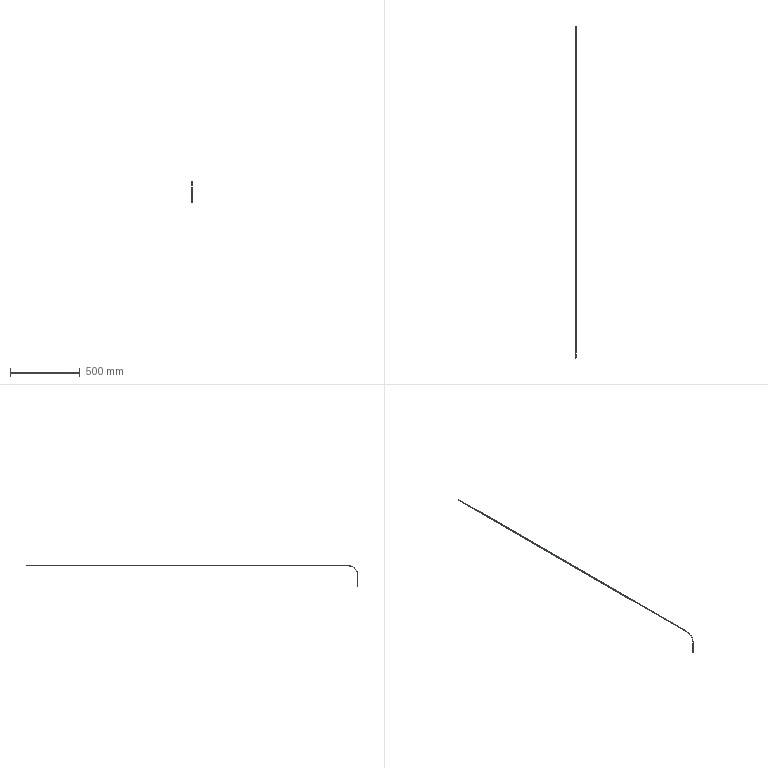Component | SolidWorks | A-SideAluminumCasingAssembly-1_C-SideSealant1-2 | 1 solid | 14 faces | box 6 x 2375.5 x 149.5 mm | volume 44871 mm3 | plane 12 | cylinder 2 | commonest cylinder face diameters 139 x1 133 x1
STEP:
#1=COLOUR_RGB('',0.7922,0.8196,0.9333);
#2=FILL_AREA_STYLE_COLOUR('',#1);
#3=FILL_AREA_STYLE('',(#2));
#4=SURFACE_STYLE_FILL_AREA(#3);
#5=SURFACE_SIDE_STYLE('',(#4));
#6=SURFACE_STYLE_USAGE(.BOTH.,#5);
#7=PRESENTATION_STYLE_ASSIGNMENT((#6));
#8=CARTESIAN_POINT('',(-0.,90.787,73.937));
#9=VERTEX_POINT('',#8);
#10=CARTESIAN_POINT('',(-0.,90.787,73.819));
#11=VERTEX_POINT('',#10);
#12=CARTESIAN_POINT('',(-0.,90.787,73.819));
#13=DIRECTION('',(0.,-0.,-1.));
#14=VECTOR('',#13,39.37);
#15=LINE('',#12,#14);
#16=EDGE_CURVE('',#9,#11,#15,.T.);
#17=ORIENTED_EDGE('',*,*,#16,.F.);
#18=CARTESIAN_POINT('',(0.,0.,73.937));
#19=VERTEX_POINT('',#18);
#20=CARTESIAN_POINT('',(0.,0.,73.937));
#21=DIRECTION('',(-0.,1.,-0.));
#22=VECTOR('',#21,39.37);
#23=LINE('',#20,#22);
#24=EDGE_CURVE('',#19,#9,#23,.T.);
#25=ORIENTED_EDGE('',*,*,#24,.F.);
#26=CARTESIAN_POINT('',(0.,0.,73.819));
#27=VERTEX_POINT('',#26);
#28=CARTESIAN_POINT('',(0.,0.,73.819));
#29=DIRECTION('',(0.,-0.,-1.));
#30=VECTOR('',#29,39.37);
#31=LINE('',#28,#30);
#32=EDGE_CURVE('',#19,#27,#31,.T.);
#33=ORIENTED_EDGE('',*,*,#32,.T.);
#34=CARTESIAN_POINT('',(0.,0.,73.819));
#35=DIRECTION('',(-0.,1.,-0.));
#36=VECTOR('',#35,39.37);
#37=LINE('',#34,#36);
#38=EDGE_CURVE('',#27,#11,#37,.T.);
#39=ORIENTED_EDGE('',*,*,#38,.T.);
#40=EDGE_LOOP('',(#17,#25,#33,#39));
#41=FACE_OUTER_BOUND('',#40,.T.);
#42=CARTESIAN_POINT('',(0.,0.,73.819));
#43=DIRECTION('',(1.,0.,0.));
#44=DIRECTION('',(-0.,1.,-0.));
#45=AXIS2_PLACEMENT_3D('',#42,#43,#44);
#46=PLANE('',#45);
#47=ADVANCED_FACE('',(#41),#46,.T.);
#48=CARTESIAN_POINT('',(-0.2362,0.,73.937));
#49=VERTEX_POINT('',#48);
#50=CARTESIAN_POINT('',(-0.2362,0.,73.819));
#51=VERTEX_POINT('',#50);
#52=CARTESIAN_POINT('',(-0.2362,0.,73.819));
#53=DIRECTION('',(0.,-0.,-1.));
#54=VECTOR('',#53,39.37);
#55=LINE('',#52,#54);
#56=EDGE_CURVE('',#49,#51,#55,.T.);
#57=ORIENTED_EDGE('',*,*,#56,.F.);
#58=CARTESIAN_POINT('',(-0.2362,90.787,73.937));
#59=VERTEX_POINT('',#58);
#60=CARTESIAN_POINT('',(-0.2362,0.,73.937));
#61=DIRECTION('',(-0.,1.,-0.));
#62=VECTOR('',#61,39.37);
#63=LINE('',#60,#62);
#64=EDGE_CURVE('',#49,#59,#63,.T.);
#65=ORIENTED_EDGE('',*,*,#64,.T.);
#66=CARTESIAN_POINT('',(-0.2362,90.787,73.819));
#67=VERTEX_POINT('',#66);
#68=CARTESIAN_POINT('',(-0.2362,90.787,73.819));
#69=DIRECTION('',(0.,-0.,-1.));
#70=VECTOR('',#69,39.37);
#71=LINE('',#68,#70);
#72=EDGE_CURVE('',#59,#67,#71,.T.);
#73=ORIENTED_EDGE('',*,*,#72,.T.);
#74=CARTESIAN_POINT('',(-0.2362,0.,73.819));
#75=DIRECTION('',(-0.,1.,-0.));
#76=VECTOR('',#75,39.37);
#77=LINE('',#74,#76);
#78=EDGE_CURVE('',#51,#67,#77,.T.);
#79=ORIENTED_EDGE('',*,*,#78,.F.);
#80=EDGE_LOOP('',(#57,#65,#73,#79));
#81=FACE_OUTER_BOUND('',#80,.T.);
#82=CARTESIAN_POINT('',(-0.2362,0.,73.819));
#83=DIRECTION('',(1.,0.,0.));
#84=DIRECTION('',(-0.,1.,-0.));
#85=AXIS2_PLACEMENT_3D('',#82,#83,#84);
#86=PLANE('',#85);
#87=ADVANCED_FACE('',(#81),#86,.F.);
#88=CARTESIAN_POINT('',(-0.1181,90.787,73.937));
#89=DIRECTION('',(-1.,-0.,-0.));
#90=VECTOR('',#89,39.37);
#91=LINE('',#88,#90);
#92=EDGE_CURVE('',#9,#59,#91,.T.);
#93=ORIENTED_EDGE('',*,*,#92,.F.);
#94=ORIENTED_EDGE('',*,*,#16,.T.);
#95=CARTESIAN_POINT('',(-0.,90.787,73.819));
#96=DIRECTION('',(-1.,-0.,-0.));
#97=VECTOR('',#96,39.37);
#98=LINE('',#95,#97);
#99=EDGE_CURVE('',#11,#67,#98,.T.);
#100=ORIENTED_EDGE('',*,*,#99,.T.);
#101=ORIENTED_EDGE('',*,*,#72,.F.);
#102=EDGE_LOOP('',(#93,#94,#100,#101));
#103=FACE_OUTER_BOUND('',#102,.T.);
#104=CARTESIAN_POINT('',(-0.,90.787,73.819));
#105=DIRECTION('',(-0.,1.,-0.));
#106=DIRECTION('',(-1.,-0.,-0.));
#107=AXIS2_PLACEMENT_3D('',#104,#105,#106);
#108=PLANE('',#107);
#109=ADVANCED_FACE('',(#103),#108,.T.);
#110=ORIENTED_EDGE('',*,*,#78,.T.);
#111=ORIENTED_EDGE('',*,*,#99,.F.);
#112=ORIENTED_EDGE('',*,*,#38,.F.);
#113=CARTESIAN_POINT('',(-0.2362,0.,73.819));
#114=DIRECTION('',(1.,0.,0.));
#115=VECTOR('',#114,39.37);
#116=LINE('',#113,#115);
#117=EDGE_CURVE('',#51,#27,#116,.T.);
#118=ORIENTED_EDGE('',*,*,#117,.F.);
#119=EDGE_LOOP('',(#110,#111,#112,#118));
#120=FACE_OUTER_BOUND('',#119,.T.);
#121=CARTESIAN_POINT('',(-0.1181,0.,73.819));
#122=DIRECTION('',(-0.,0.,1.));
#123=DIRECTION('',(1.,0.,0.));
#124=AXIS2_PLACEMENT_3D('',#121,#122,#123);
#125=PLANE('',#124);
#126=ADVANCED_FACE('',(#120),#125,.F.);
#127=ORIENTED_EDGE('',*,*,#64,.F.);
#128=CARTESIAN_POINT('',(-0.1181,0.,73.937));
#129=DIRECTION('',(1.,0.,0.));
#130=VECTOR('',#129,39.37);
#131=LINE('',#128,#130);
#132=EDGE_CURVE('',#49,#19,#131,.T.);
#133=ORIENTED_EDGE('',*,*,#132,.T.);
#134=ORIENTED_EDGE('',*,*,#24,.T.);
#135=ORIENTED_EDGE('',*,*,#92,.T.);
#136=EDGE_LOOP('',(#127,#133,#134,#135));
#137=FACE_OUTER_BOUND('',#136,.T.);
#138=CARTESIAN_POINT('',(-0.1181,0.,73.937));
#139=DIRECTION('',(-0.,0.,1.));
#140=DIRECTION('',(1.,0.,0.));
#141=AXIS2_PLACEMENT_3D('',#138,#139,#140);
#142=PLANE('',#141);
#143=ADVANCED_FACE('',(#137),#142,.T.);
#144=CARTESIAN_POINT('',(0.,-2.618,71.201));
#145=VERTEX_POINT('',#144);
#146=CARTESIAN_POINT('',(0.,-2.736,71.201));
#147=VERTEX_POINT('',#146);
#148=CARTESIAN_POINT('',(0.,-2.736,71.201));
#149=DIRECTION('',(0.,-1.,0.));
#150=VECTOR('',#149,39.37);
#151=LINE('',#148,#150);
#152=EDGE_CURVE('',#145,#147,#151,.T.);
#153=ORIENTED_EDGE('',*,*,#152,.F.);
#154=CARTESIAN_POINT('',(0.,0.,71.201));
#155=DIRECTION('',(1.,0.,0.));
#156=DIRECTION('',(-0.,0.,1.));
#157=AXIS2_PLACEMENT_3D('',#154,#155,#156);
#158=CIRCLE('',#157,2.618);
#159=EDGE_CURVE('',#27,#145,#158,.T.);
#160=ORIENTED_EDGE('',*,*,#159,.F.);
#161=ORIENTED_EDGE('',*,*,#32,.F.);
#162=CARTESIAN_POINT('',(0.,0.,71.201));
#163=DIRECTION('',(1.,0.,0.));
#164=DIRECTION('',(-0.,0.,1.));
#165=AXIS2_PLACEMENT_3D('',#162,#163,#164);
#166=CIRCLE('',#165,2.736);
#167=EDGE_CURVE('',#19,#147,#166,.T.);
#168=ORIENTED_EDGE('',*,*,#167,.T.);
#169=EDGE_LOOP('',(#153,#160,#161,#168));
#170=FACE_OUTER_BOUND('',#169,.T.);
#171=CARTESIAN_POINT('',(0.,0.,71.201));
#172=DIRECTION('',(1.,0.,0.));
#173=DIRECTION('',(0.,-0.,-1.));
#174=AXIS2_PLACEMENT_3D('',#171,#172,#173);
#175=PLANE('',#174);
#176=ADVANCED_FACE('',(#170),#175,.T.);
#177=CARTESIAN_POINT('',(-0.2362,-2.618,71.201));
#178=VERTEX_POINT('',#177);
#179=CARTESIAN_POINT('',(-0.2362,0.,71.201));
#180=DIRECTION('',(-1.,-0.,-0.));
#181=DIRECTION('',(-0.,0.,1.));
#182=AXIS2_PLACEMENT_3D('',#179,#180,#181);
#183=CIRCLE('',#182,2.618);
#184=EDGE_CURVE('',#178,#51,#183,.T.);
#185=ORIENTED_EDGE('',*,*,#184,.F.);
#186=CARTESIAN_POINT('',(-0.2362,-2.736,71.201));
#187=VERTEX_POINT('',#186);
#188=CARTESIAN_POINT('',(-0.2362,-2.618,71.201));
#189=DIRECTION('',(0.,-1.,0.));
#190=VECTOR('',#189,39.37);
#191=LINE('',#188,#190);
#192=EDGE_CURVE('',#178,#187,#191,.T.);
#193=ORIENTED_EDGE('',*,*,#192,.T.);
#194=CARTESIAN_POINT('',(-0.2362,0.,71.201));
#195=DIRECTION('',(-1.,-0.,-0.));
#196=DIRECTION('',(-0.,0.,1.));
#197=AXIS2_PLACEMENT_3D('',#194,#195,#196);
#198=CIRCLE('',#197,2.736);
#199=EDGE_CURVE('',#187,#49,#198,.T.);
#200=ORIENTED_EDGE('',*,*,#199,.T.);
#201=ORIENTED_EDGE('',*,*,#56,.T.);
#202=EDGE_LOOP('',(#185,#193,#200,#201));
#203=FACE_OUTER_BOUND('',#202,.T.);
#204=CARTESIAN_POINT('',(-0.2362,0.,71.201));
#205=DIRECTION('',(1.,0.,0.));
#206=DIRECTION('',(0.,-0.,-1.));
#207=AXIS2_PLACEMENT_3D('',#204,#205,#206);
#208=PLANE('',#207);
#209=ADVANCED_FACE('',(#203),#208,.F.);
#210=ORIENTED_EDGE('',*,*,#132,.F.);
#211=ORIENTED_EDGE('',*,*,#199,.F.);
#212=CARTESIAN_POINT('',(0.,-2.736,71.201));
#213=DIRECTION('',(1.,0.,0.));
#214=VECTOR('',#213,39.37);
#215=LINE('',#212,#214);
#216=EDGE_CURVE('',#187,#147,#215,.T.);
#217=ORIENTED_EDGE('',*,*,#216,.T.);
#218=ORIENTED_EDGE('',*,*,#167,.F.);
#219=EDGE_LOOP('',(#210,#211,#217,#218));
#220=FACE_OUTER_BOUND('',#219,.T.);
#221=CARTESIAN_POINT('',(-0.2362,0.,71.201));
#222=DIRECTION('',(-1.,-0.,-0.));
#223=DIRECTION('',(0.,-1.,0.));
#224=AXIS2_PLACEMENT_3D('',#221,#222,#223);
#225=CYLINDRICAL_SURFACE('',#224,2.736);
#226=ADVANCED_FACE('',(#220),#225,.T.);
#227=ORIENTED_EDGE('',*,*,#117,.T.);
#228=ORIENTED_EDGE('',*,*,#159,.T.);
#229=CARTESIAN_POINT('',(0.,-2.618,71.201));
#230=DIRECTION('',(-1.,-0.,-0.));
#231=VECTOR('',#230,39.37);
#232=LINE('',#229,#231);
#233=EDGE_CURVE('',#145,#178,#232,.T.);
#234=ORIENTED_EDGE('',*,*,#233,.T.);
#235=ORIENTED_EDGE('',*,*,#184,.T.);
#236=EDGE_LOOP('',(#227,#228,#234,#235));
#237=FACE_OUTER_BOUND('',#236,.T.);
#238=CARTESIAN_POINT('',(-0.2362,0.,71.201));
#239=DIRECTION('',(-1.,-0.,-0.));
#240=DIRECTION('',(0.,-1.,0.));
#241=AXIS2_PLACEMENT_3D('',#238,#239,#240);
#242=CYLINDRICAL_SURFACE('',#241,2.618);
#243=ADVANCED_FACE('',(#237),#242,.F.);
#244=ORIENTED_EDGE('',*,*,#192,.F.);
#245=CARTESIAN_POINT('',(-0.2362,-2.618,68.051));
#246=VERTEX_POINT('',#245);
#247=CARTESIAN_POINT('',(-0.2362,-2.618,68.051));
#248=DIRECTION('',(0.,-0.,-1.));
#249=VECTOR('',#248,39.37);
#250=LINE('',#247,#249);
#251=EDGE_CURVE('',#178,#246,#250,.T.);
#252=ORIENTED_EDGE('',*,*,#251,.T.);
#253=CARTESIAN_POINT('',(-0.2362,-2.736,68.051));
#254=VERTEX_POINT('',#253);
#255=CARTESIAN_POINT('',(-0.2362,-2.736,68.051));
#256=DIRECTION('',(-0.,1.,-0.));
#257=VECTOR('',#256,39.37);
#258=LINE('',#255,#257);
#259=EDGE_CURVE('',#254,#246,#258,.T.);
#260=ORIENTED_EDGE('',*,*,#259,.F.);
#261=CARTESIAN_POINT('',(-0.2362,-2.736,73.819));
#262=DIRECTION('',(0.,-0.,-1.));
#263=VECTOR('',#262,39.37);
#264=LINE('',#261,#263);
#265=EDGE_CURVE('',#187,#254,#264,.T.);
#266=ORIENTED_EDGE('',*,*,#265,.F.);
#267=EDGE_LOOP('',(#244,#252,#260,#266));
#268=FACE_OUTER_BOUND('',#267,.T.);
#269=CARTESIAN_POINT('',(-0.2362,-2.736,68.051));
#270=DIRECTION('',(1.,0.,0.));
#271=DIRECTION('',(0.,-0.,-1.));
#272=AXIS2_PLACEMENT_3D('',#269,#270,#271);
#273=PLANE('',#272);
#274=ADVANCED_FACE('',(#268),#273,.F.);
#275=ORIENTED_EDGE('',*,*,#152,.T.);
#276=CARTESIAN_POINT('',(0.,-2.736,68.051));
#277=VERTEX_POINT('',#276);
#278=CARTESIAN_POINT('',(0.,-2.736,73.819));
#279=DIRECTION('',(-0.,0.,1.));
#280=VECTOR('',#279,39.37);
#281=LINE('',#278,#280);
#282=EDGE_CURVE('',#277,#147,#281,.T.);
#283=ORIENTED_EDGE('',*,*,#282,.F.);
#284=CARTESIAN_POINT('',(0.,-2.618,68.051));
#285=VERTEX_POINT('',#284);
#286=CARTESIAN_POINT('',(0.,-2.736,68.051));
#287=DIRECTION('',(-0.,1.,-0.));
#288=VECTOR('',#287,39.37);
#289=LINE('',#286,#288);
#290=EDGE_CURVE('',#277,#285,#289,.T.);
#291=ORIENTED_EDGE('',*,*,#290,.T.);
#292=CARTESIAN_POINT('',(0.,-2.618,73.819));
#293=DIRECTION('',(-0.,0.,1.));
#294=VECTOR('',#293,39.37);
#295=LINE('',#292,#294);
#296=EDGE_CURVE('',#285,#145,#295,.T.);
#297=ORIENTED_EDGE('',*,*,#296,.T.);
#298=EDGE_LOOP('',(#275,#283,#291,#297));
#299=FACE_OUTER_BOUND('',#298,.T.);
#300=CARTESIAN_POINT('',(0.,-2.736,73.819));
#301=DIRECTION('',(-1.,-0.,-0.));
#302=DIRECTION('',(-0.,0.,1.));
#303=AXIS2_PLACEMENT_3D('',#300,#301,#302);
#304=PLANE('',#303);
#305=ADVANCED_FACE('',(#299),#304,.F.);
#306=ORIENTED_EDGE('',*,*,#216,.F.);
#307=ORIENTED_EDGE('',*,*,#265,.T.);
#308=CARTESIAN_POINT('',(-0.1181,-2.736,68.051));
#309=DIRECTION('',(1.,0.,0.));
#310=VECTOR('',#309,39.37);
#311=LINE('',#308,#310);
#312=EDGE_CURVE('',#254,#277,#311,.T.);
#313=ORIENTED_EDGE('',*,*,#312,.T.);
#314=ORIENTED_EDGE('',*,*,#282,.T.);
#315=EDGE_LOOP('',(#306,#307,#313,#314));
#316=FACE_OUTER_BOUND('',#315,.T.);
#317=CARTESIAN_POINT('',(-0.1181,-2.736,73.819));
#318=DIRECTION('',(-0.,1.,-0.));
#319=DIRECTION('',(0.,-0.,-1.));
#320=AXIS2_PLACEMENT_3D('',#317,#318,#319);
#321=PLANE('',#320);
#322=ADVANCED_FACE('',(#316),#321,.F.);
#323=ORIENTED_EDGE('',*,*,#251,.F.);
#324=ORIENTED_EDGE('',*,*,#233,.F.);
#325=ORIENTED_EDGE('',*,*,#296,.F.);
#326=CARTESIAN_POINT('',(0.,-2.618,68.051));
#327=DIRECTION('',(1.,0.,0.));
#328=VECTOR('',#327,39.37);
#329=LINE('',#326,#328);
#330=EDGE_CURVE('',#246,#285,#329,.T.);
#331=ORIENTED_EDGE('',*,*,#330,.F.);
#332=EDGE_LOOP('',(#323,#324,#325,#331));
#333=FACE_OUTER_BOUND('',#332,.T.);
#334=CARTESIAN_POINT('',(-0.1181,-2.618,73.819));
#335=DIRECTION('',(-0.,1.,-0.));
#336=DIRECTION('',(0.,-0.,-1.));
#337=AXIS2_PLACEMENT_3D('',#334,#335,#336);
#338=PLANE('',#337);
#339=ADVANCED_FACE('',(#333),#338,.T.);
#340=ORIENTED_EDGE('',*,*,#330,.T.);
#341=ORIENTED_EDGE('',*,*,#290,.F.);
#342=ORIENTED_EDGE('',*,*,#312,.F.);
#343=ORIENTED_EDGE('',*,*,#259,.T.);
#344=EDGE_LOOP('',(#340,#341,#342,#343));
#345=FACE_OUTER_BOUND('',#344,.T.);
#346=CARTESIAN_POINT('',(0.,-2.736,68.051));
#347=DIRECTION('',(-0.,0.,1.));
#348=DIRECTION('',(-0.,1.,-0.));
#349=AXIS2_PLACEMENT_3D('',#346,#347,#348);
#350=PLANE('',#349);
#351=ADVANCED_FACE('',(#345),#350,.F.);
#352=CLOSED_SHELL('',(#47,#87,#109,#126,#143,#176,#209,#226,#243,#274,#305,#322,#339,#351));
#353=MANIFOLD_SOLID_BREP('',#352);
#354=STYLED_ITEM('',(#7),#353);
#355=(LENGTH_UNIT()NAMED_UNIT(*)SI_UNIT($,.METRE.));
#356=LENGTH_MEASURE_WITH_UNIT(LENGTH_MEASURE(0.0254),#355);
#357=DIMENSIONAL_EXPONENTS(1.,0.,0.,0.,0.,0.,0.);
#358=(CONVERSION_BASED_UNIT('',#356)LENGTH_UNIT()NAMED_UNIT(#357));
#359=UNCERTAINTY_MEASURE_WITH_UNIT(LENGTH_MEASURE(0.00001),#358,'','');
#360=(NAMED_UNIT(*)PLANE_ANGLE_UNIT()SI_UNIT($,.RADIAN.));
#361=(NAMED_UNIT(*)SI_UNIT($,.STERADIAN.)SOLID_ANGLE_UNIT());
#362=(GEOMETRIC_REPRESENTATION_CONTEXT(3)GLOBAL_UNCERTAINTY_ASSIGNED_CONTEXT((#359))GLOBAL_UNIT_ASSIGNED_CONTEXT((#358,#360,#361))REPRESENTATION_CONTEXT('',''));
#363=MECHANICAL_DESIGN_GEOMETRIC_PRESENTATION_REPRESENTATION('',(#354),#362);
#364=CARTESIAN_POINT('',(0.,0.,0.));
#365=DIRECTION('',(0.,0.,1.));
#366=DIRECTION('',(1.,0.,0.));
#367=AXIS2_PLACEMENT_3D('',#364,#365,#366);
#368=(LENGTH_UNIT()NAMED_UNIT(*)SI_UNIT($,.METRE.));
#369=LENGTH_MEASURE_WITH_UNIT(LENGTH_MEASURE(0.0254),#368);
#370=DIMENSIONAL_EXPONENTS(1.,0.,0.,0.,0.,0.,0.);
#371=(CONVERSION_BASED_UNIT('',#369)LENGTH_UNIT()NAMED_UNIT(#370));
#372=UNCERTAINTY_MEASURE_WITH_UNIT(LENGTH_MEASURE(0.00001),#371,'','');
#373=(NAMED_UNIT(*)PLANE_ANGLE_UNIT()SI_UNIT($,.RADIAN.));
#374=(NAMED_UNIT(*)SI_UNIT($,.STERADIAN.)SOLID_ANGLE_UNIT());
#375=(GEOMETRIC_REPRESENTATION_CONTEXT(3)GLOBAL_UNCERTAINTY_ASSIGNED_CONTEXT((#372))GLOBAL_UNIT_ASSIGNED_CONTEXT((#371,#373,#374))REPRESENTATION_CONTEXT('',''));
#376=ADVANCED_BREP_SHAPE_REPRESENTATION('',(#353,#367),#375);
#377=PRESENTATION_LAYER_ASSIGNMENT('','',(#354));